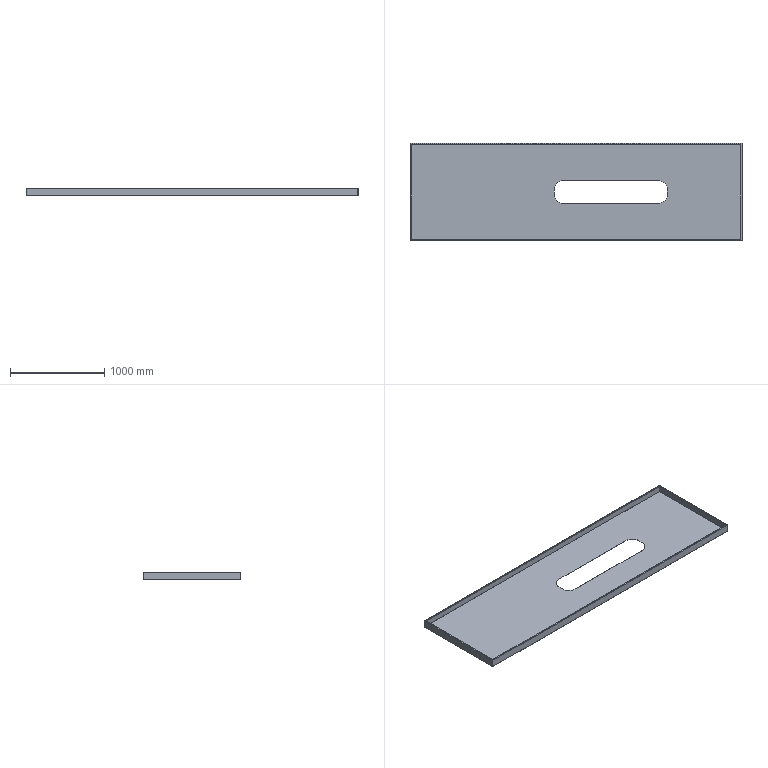Component | NX | DB4_1 | 1 solid | 24 faces | volume 6264138 mm3 | plane 20 | cylinder 4 | commonest cylinder face diameters 200 x4